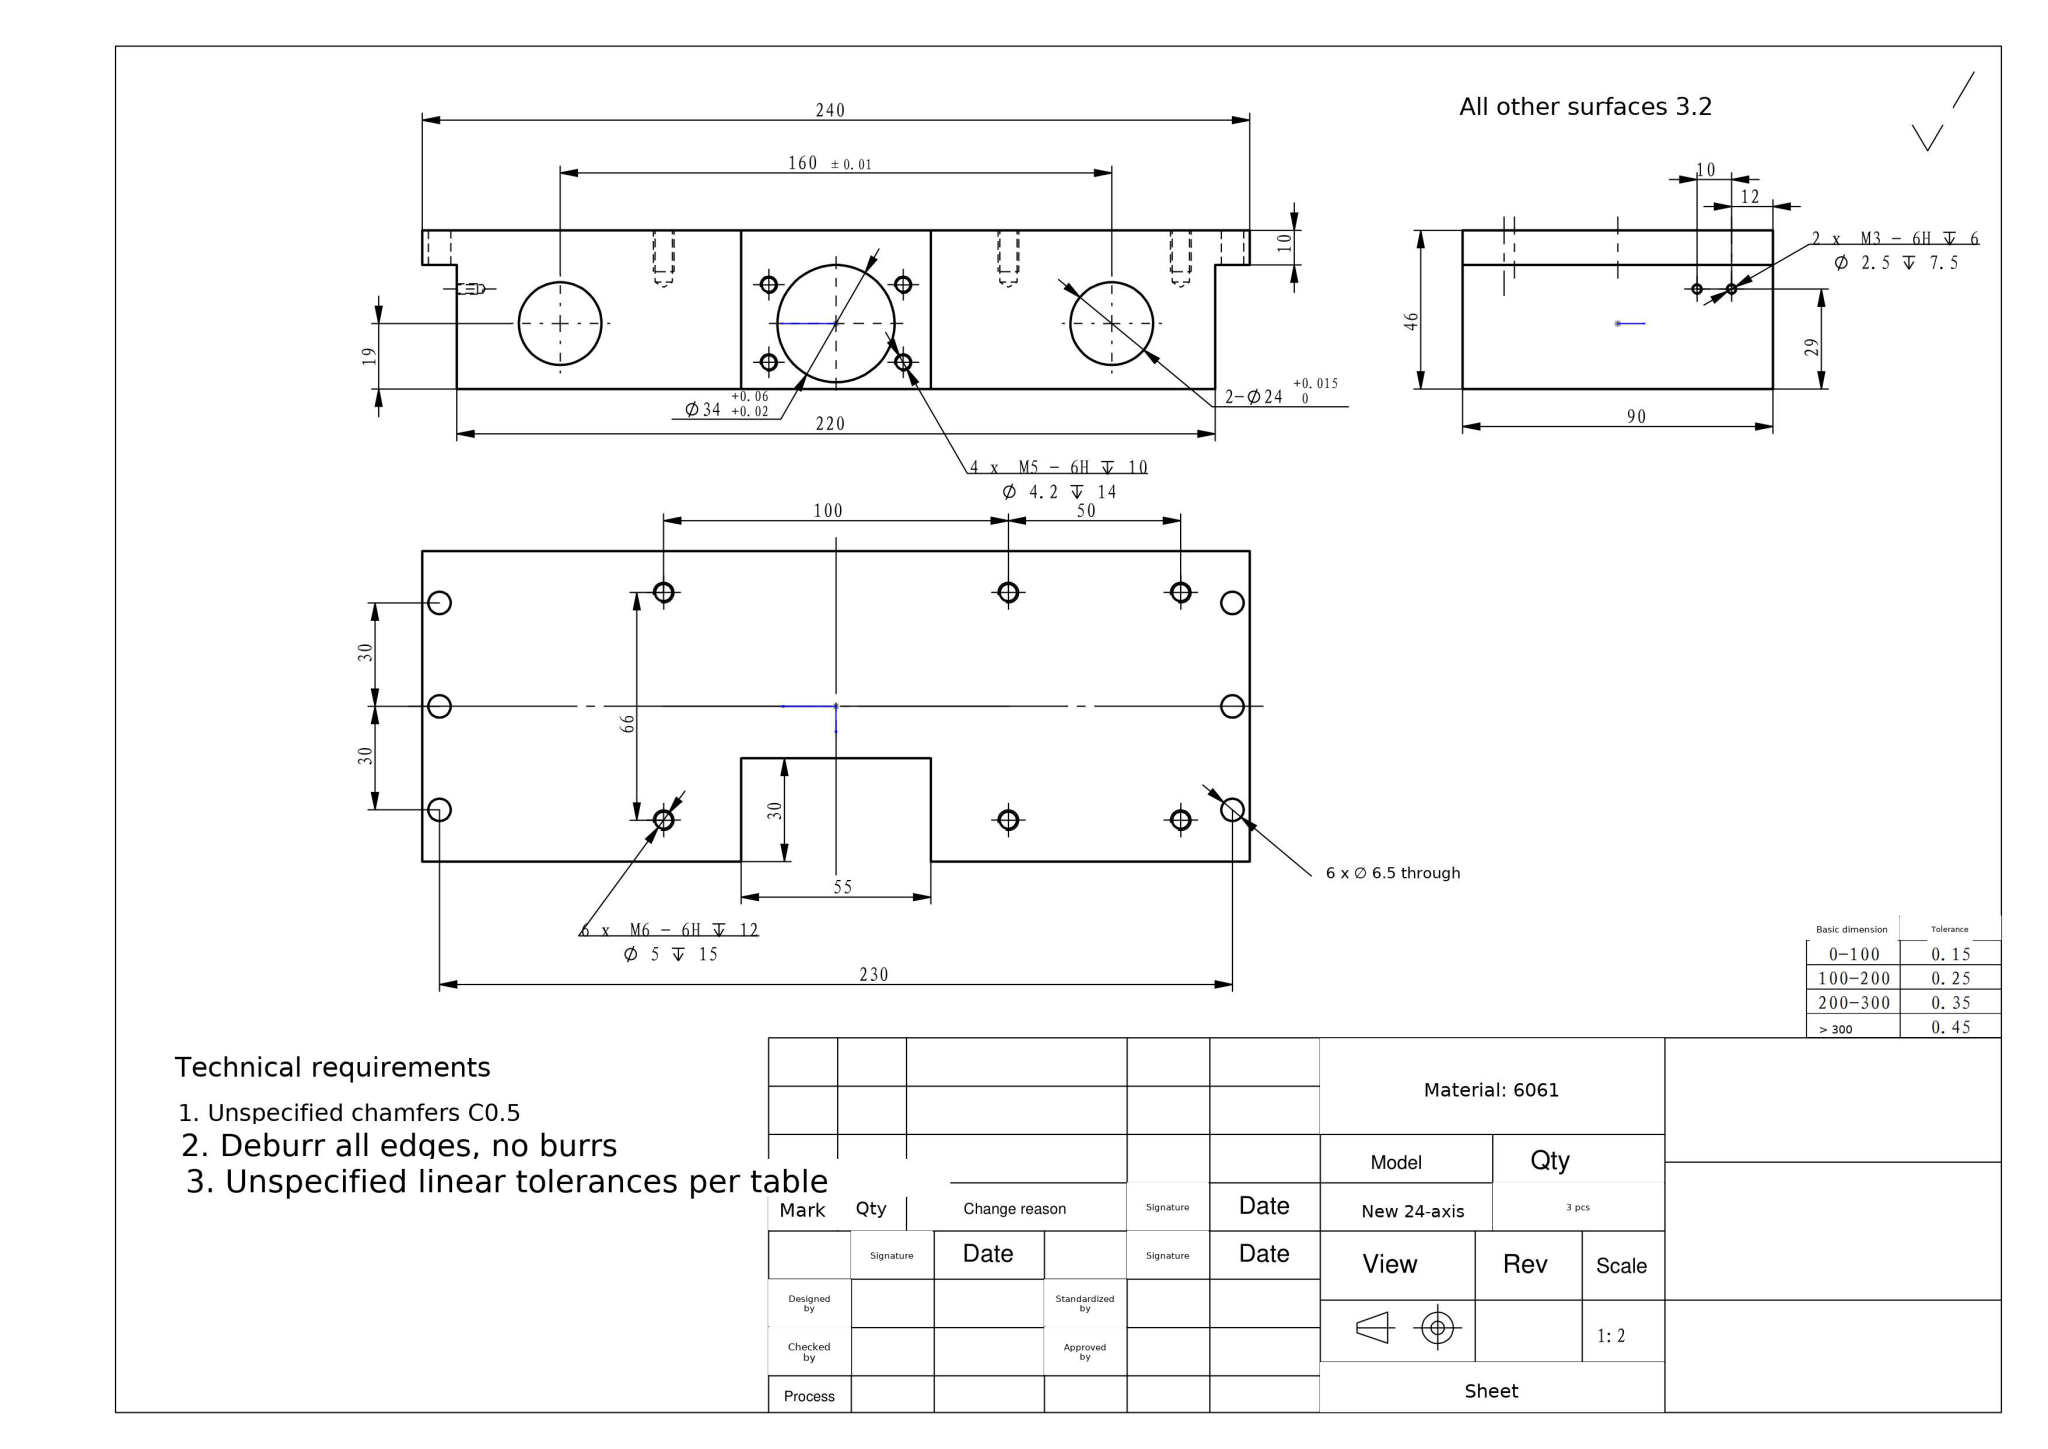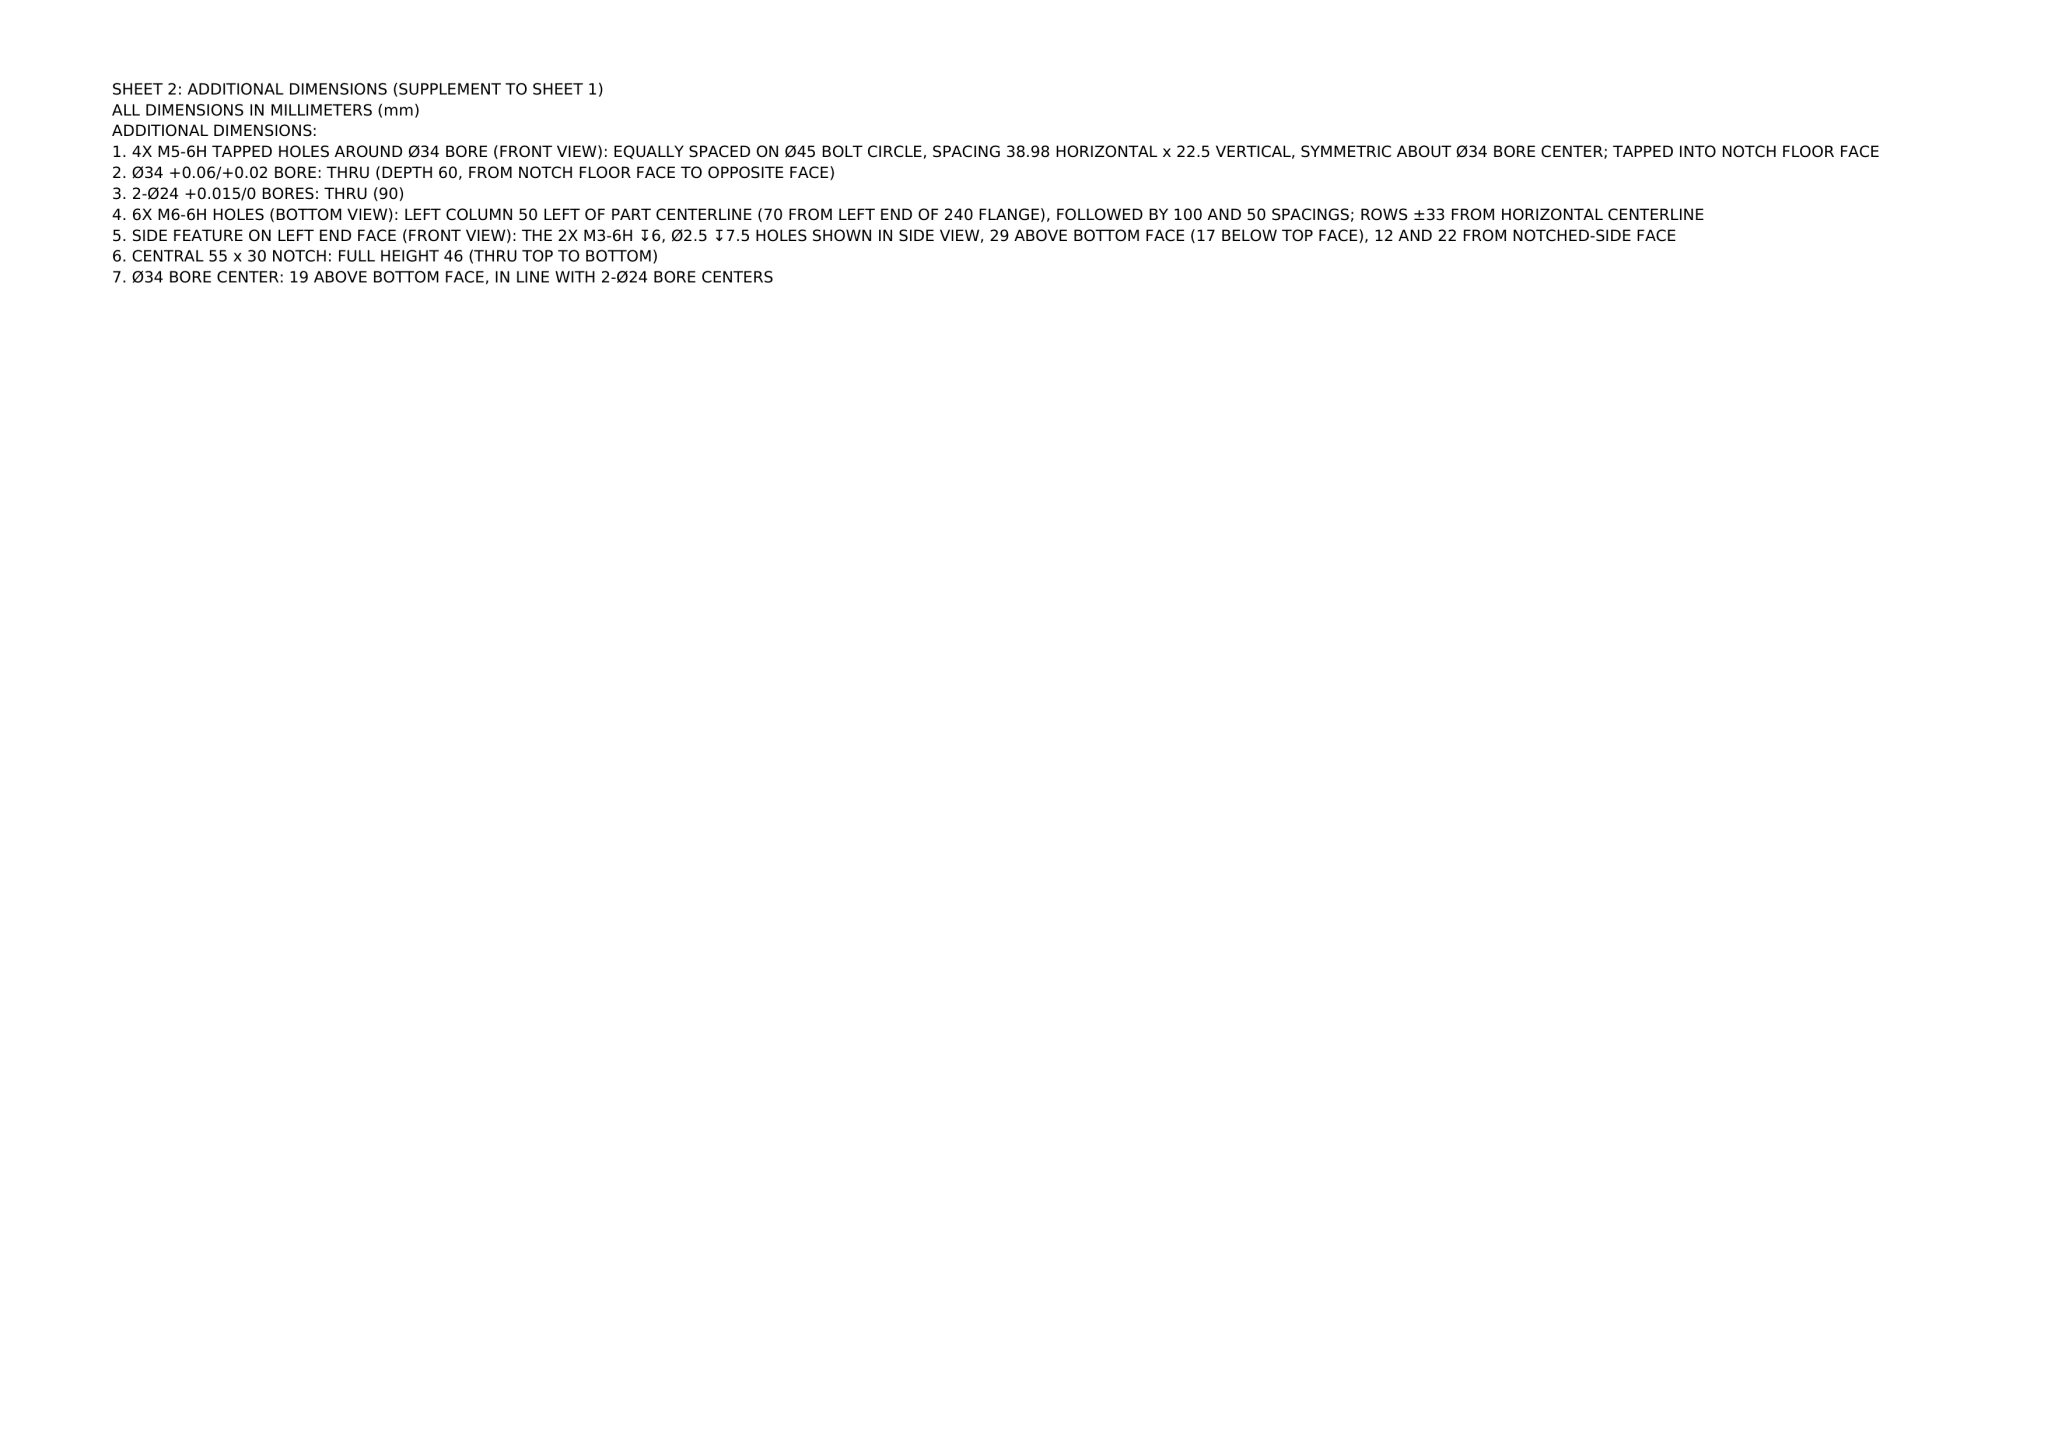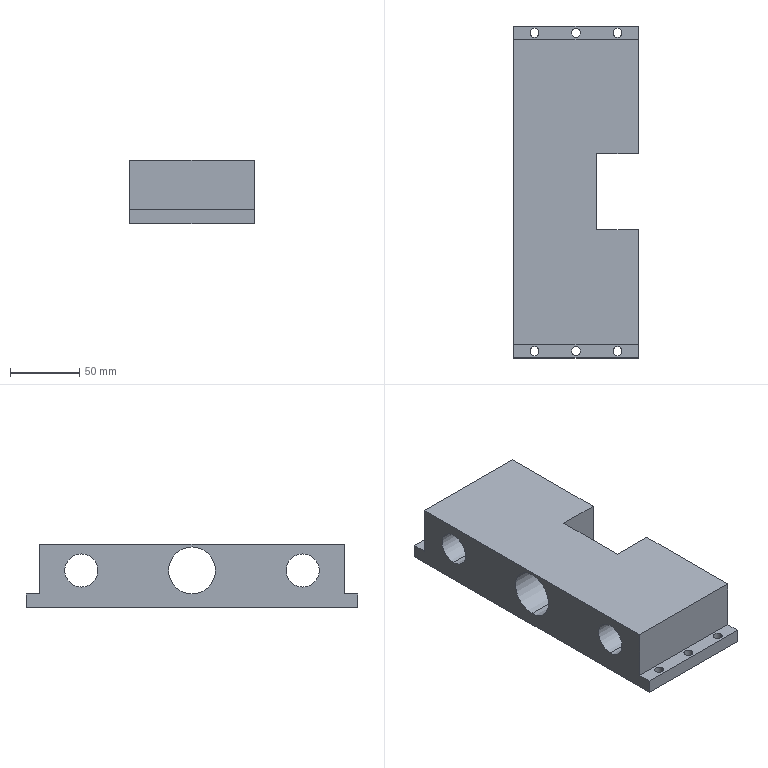Part | NX | mm | 1 solid | 80 faces | box 90 x 240 x 46 mm | volume 712302 mm3 | cylinder 42 | cone 24 | plane 14 | commonest cylinder face diameters 6.5 x12 5 x12 4.2 x8 2.5 x4 24 x4 34 x2